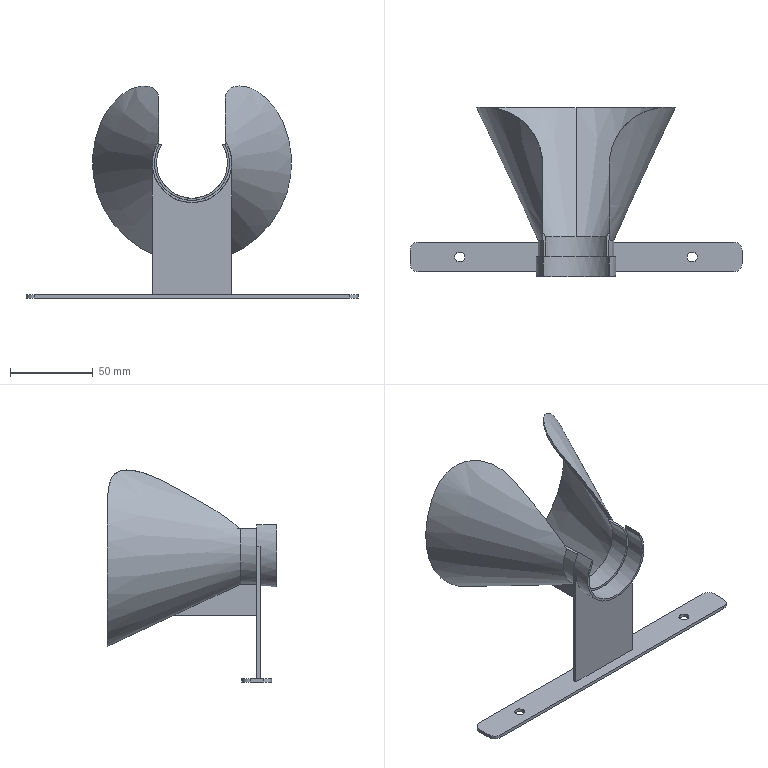Component | SolidWorks | DoughGuideFunnel-1 | 2 solids | 44 faces | volume 52371 mm3 | plane 26 | cylinder 14 | cone 4 | commonest cylinder face diameters 6 x4 10 x4 45.391 x2 70 x2 48 x1 42.842 x1